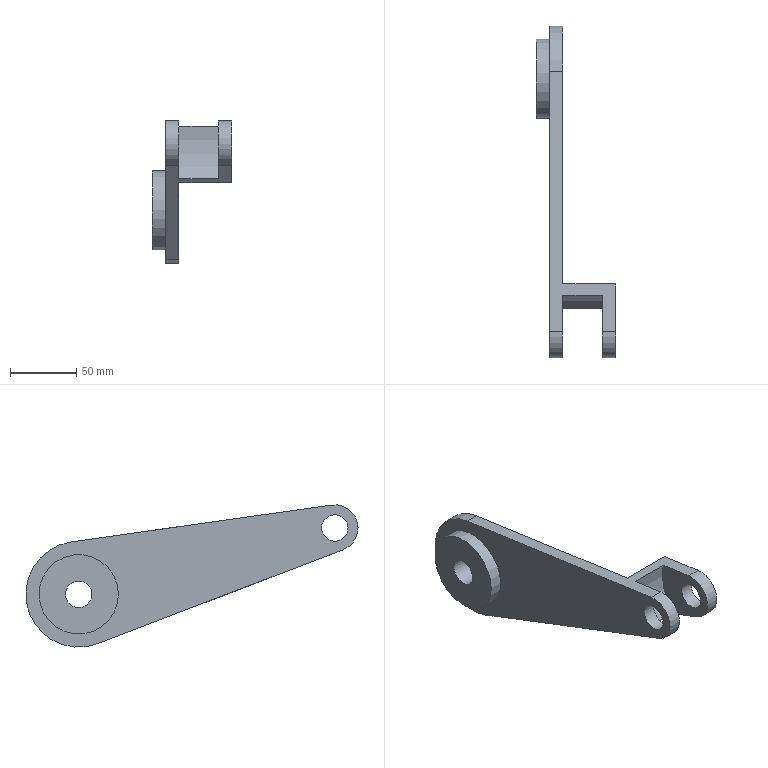Component | NX | CCJ-007 | 1 solid | 17 faces | volume 191325 mm3 | cylinder 9 | plane 8 | commonest cylinder face diameters 20 x3 35 x2 80 x1 116.418 x1 100 x1 60 x1